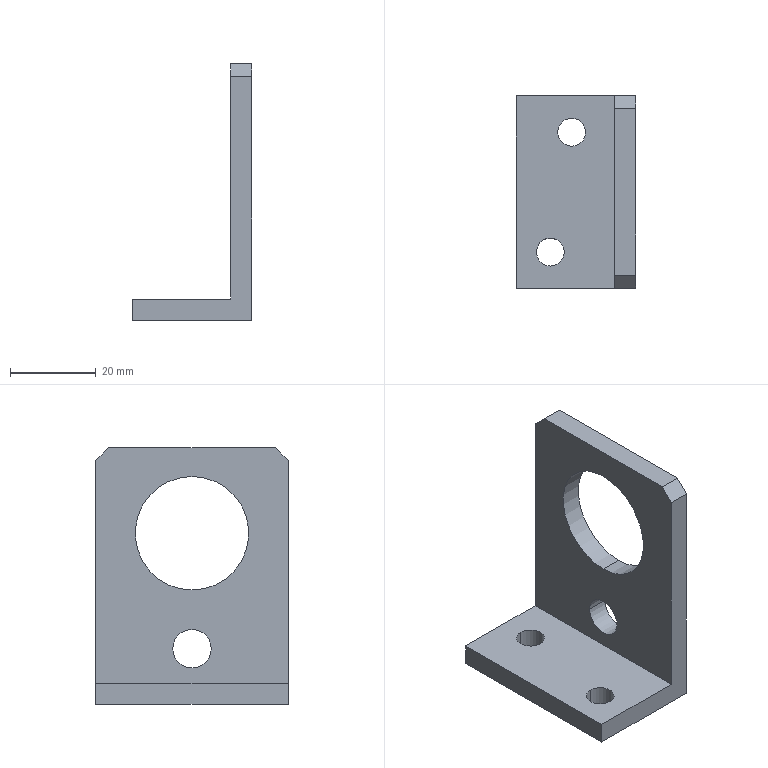Component | SolidWorks | DC-Motor-113-1 | 1 solid | 18 faces | box 28 x 45 x 60 mm | volume 15222 mm3 | plane 10 | cylinder 8 | commonest cylinder face diameters 6.5 x4 9 x2 26.5 x2
build123d program:
from build123d import *

# Parameters (mm, degrees)
BOSS_EXTRUDE1_DEPTH          = 22.5
SKETCH4_R                    = 13.25
CUT_EXTRUDE1_DEPTH           = 42
CHAMFER1_SIZE                = 3
F_6_5_6_5_DIAMETER_HOLE1_D   = 6.5
F_9_0_9_DIAMETER_HOLE1_D     = 9
F_9_0_9_DIAMETER_HOLE1_DEPTH = 12.4
F_9_0_9_DIAMETER_HOLE1_TIP   = 2.704


with BuildPart() as part:
    # Sketch1 → Boss-Extrude1 (new, symmetric)
    with BuildSketch(Plane.XY):
        Polygon((0, 60), (0, 0), (28, 0), (28, 5), (5, 5), (5, 60), align=None)
    extrude(amount=BOSS_EXTRUDE1_DEPTH, both=True)

    # Sketch4 → Cut-Extrude1 (cut)
    with BuildSketch(Plane(origin=(5, 0, 0), x_dir=(0, 0, -1), z_dir=(1, 0, 0))):
        with Locations(Location((0, 40, 0), (0, 0, 90))):
            Circle(SKETCH4_R)
    extrude(amount=-CUT_EXTRUDE1_DEPTH, mode=Mode.SUBTRACT)

    # Chamfer1
    chamfer1_edges = [part.edges().sort_by_distance(p)[0] for p in [
        (2.5, 60, 22.5),
        (2.5, 60, -22.5),
    ]]
    chamfer(chamfer1_edges, length=CHAMFER1_SIZE)

    # 6.5 _6.5_ Diameter Hole1 (through all)
    with Locations(Plane(origin=(0, 5, 0), x_dir=(1, 0, 0), z_dir=(0, 1, 0))):
        with Locations((20, 14), (15, -14)):
            Hole(F_6_5_6_5_DIAMETER_HOLE1_D / 2)

    # 9.0 _9_ Diameter Hole1
    with Locations(Plane(origin=(5, 0, 0), x_dir=(0, 0, -1), z_dir=(1, 0, 0))):
        with Locations((0, 13)):
            Hole(F_9_0_9_DIAMETER_HOLE1_D / 2, depth=F_9_0_9_DIAMETER_HOLE1_DEPTH)
            with Locations((0, 0, -(F_9_0_9_DIAMETER_HOLE1_DEPTH + F_9_0_9_DIAMETER_HOLE1_TIP / 2))):  # 118° drill point
                Cone(0, F_9_0_9_DIAMETER_HOLE1_D / 2, F_9_0_9_DIAMETER_HOLE1_TIP, mode=Mode.SUBTRACT)


solid = part.part

# Placed as in the assembly
solid = solid.moved(Location((-459.792, 14.301, -420), (-90, 0, 180)))
STEP:
#1=CARTESIAN_POINT('',(-18.102,0.7402,-16.024));
#2=VERTEX_POINT('',#1);
#3=CARTESIAN_POINT('',(-18.102,0.3859,-16.024));
#4=VERTEX_POINT('',#3);
#5=CARTESIAN_POINT('',(-18.102,0.563,-16.024));
#6=DIRECTION('',(-1.,-0.,-0.));
#7=DIRECTION('',(0.,-0.,1.));
#8=AXIS2_PLACEMENT_3D('',#5,#6,#7);
#9=CIRCLE('',#8,0.1772);
#10=EDGE_CURVE('',#2,#4,#9,.T.);
#11=ORIENTED_EDGE('',*,*,#10,.F.);
#12=CARTESIAN_POINT('',(-18.299,0.7402,-16.024));
#13=VERTEX_POINT('',#12);
#14=CARTESIAN_POINT('',(-18.299,0.7402,-16.024));
#15=DIRECTION('',(-1.,-0.,-0.));
#16=VECTOR('',#15,39.37);
#17=LINE('',#14,#16);
#18=EDGE_CURVE('',#2,#13,#17,.T.);
#19=ORIENTED_EDGE('',*,*,#18,.T.);
#20=CARTESIAN_POINT('',(-18.299,0.3859,-16.024));
#21=VERTEX_POINT('',#20);
#22=CARTESIAN_POINT('',(-18.299,0.563,-16.024));
#23=DIRECTION('',(-1.,-0.,-0.));
#24=DIRECTION('',(0.,-1.,0.));
#25=AXIS2_PLACEMENT_3D('',#22,#23,#24);
#26=CIRCLE('',#25,0.1772);
#27=EDGE_CURVE('',#13,#21,#26,.T.);
#28=ORIENTED_EDGE('',*,*,#27,.T.);
#29=CARTESIAN_POINT('',(-18.299,0.3859,-16.024));
#30=DIRECTION('',(-1.,-0.,-0.));
#31=VECTOR('',#30,39.37);
#32=LINE('',#29,#31);
#33=EDGE_CURVE('',#4,#21,#32,.T.);
#34=ORIENTED_EDGE('',*,*,#33,.F.);
#35=EDGE_LOOP('',(#11,#19,#28,#34));
#36=FACE_OUTER_BOUND('',#35,.T.);
#37=CARTESIAN_POINT('',(-18.299,0.563,-16.024));
#38=DIRECTION('',(-1.,-0.,-0.));
#39=DIRECTION('',(0.,-1.,0.));
#40=AXIS2_PLACEMENT_3D('',#37,#38,#39);
#41=CYLINDRICAL_SURFACE('',#40,0.1772);
#42=ADVANCED_FACE('',(#36),#41,.F.);
#43=CARTESIAN_POINT('',(-18.889,-0.1161,-16.535));
#44=VERTEX_POINT('',#43);
#45=CARTESIAN_POINT('',(-18.889,0.1398,-16.535));
#46=VERTEX_POINT('',#45);
#47=CARTESIAN_POINT('',(-18.889,0.01186,-16.535));
#48=DIRECTION('',(-0.,-0.,1.));
#49=DIRECTION('',(0.,1.,0.));
#50=AXIS2_PLACEMENT_3D('',#47,#48,#49);
#51=CIRCLE('',#50,0.128);
#52=EDGE_CURVE('',#44,#46,#51,.T.);
#53=ORIENTED_EDGE('',*,*,#52,.F.);
#54=CARTESIAN_POINT('',(-18.889,-0.1161,-16.339));
#55=VERTEX_POINT('',#54);
#56=CARTESIAN_POINT('',(-18.889,-0.1161,-16.339));
#57=DIRECTION('',(-0.,-0.,1.));
#58=VECTOR('',#57,39.37);
#59=LINE('',#56,#58);
#60=EDGE_CURVE('',#44,#55,#59,.T.);
#61=ORIENTED_EDGE('',*,*,#60,.T.);
#62=CARTESIAN_POINT('',(-18.889,0.1398,-16.339));
#63=VERTEX_POINT('',#62);
#64=CARTESIAN_POINT('',(-18.889,0.01186,-16.339));
#65=DIRECTION('',(-0.,-0.,1.));
#66=DIRECTION('',(0.,1.,0.));
#67=AXIS2_PLACEMENT_3D('',#64,#65,#66);
#68=CIRCLE('',#67,0.128);
#69=EDGE_CURVE('',#55,#63,#68,.T.);
#70=ORIENTED_EDGE('',*,*,#69,.T.);
#71=CARTESIAN_POINT('',(-18.889,0.1398,-16.339));
#72=DIRECTION('',(-0.,-0.,1.));
#73=VECTOR('',#72,39.37);
#74=LINE('',#71,#73);
#75=EDGE_CURVE('',#46,#63,#74,.T.);
#76=ORIENTED_EDGE('',*,*,#75,.F.);
#77=EDGE_LOOP('',(#53,#61,#70,#76));
#78=FACE_OUTER_BOUND('',#77,.T.);
#79=CARTESIAN_POINT('',(-18.889,0.01186,-16.339));
#80=DIRECTION('',(-0.,-0.,1.));
#81=DIRECTION('',(0.,1.,0.));
#82=AXIS2_PLACEMENT_3D('',#79,#80,#81);
#83=CYLINDRICAL_SURFACE('',#82,0.128);
#84=ADVANCED_FACE('',(#78),#83,.F.);
#85=CARTESIAN_POINT('',(-18.693,0.9863,-16.535));
#86=VERTEX_POINT('',#85);
#87=CARTESIAN_POINT('',(-18.693,1.242,-16.535));
#88=VERTEX_POINT('',#87);
#89=CARTESIAN_POINT('',(-18.693,1.114,-16.535));
#90=DIRECTION('',(-0.,-0.,1.));
#91=DIRECTION('',(0.,1.,0.));
#92=AXIS2_PLACEMENT_3D('',#89,#90,#91);
#93=CIRCLE('',#92,0.128);
#94=EDGE_CURVE('',#86,#88,#93,.T.);
#95=ORIENTED_EDGE('',*,*,#94,.F.);
#96=CARTESIAN_POINT('',(-18.693,0.9863,-16.339));
#97=VERTEX_POINT('',#96);
#98=CARTESIAN_POINT('',(-18.693,0.9863,-16.339));
#99=DIRECTION('',(-0.,-0.,1.));
#100=VECTOR('',#99,39.37);
#101=LINE('',#98,#100);
#102=EDGE_CURVE('',#86,#97,#101,.T.);
#103=ORIENTED_EDGE('',*,*,#102,.T.);
#104=CARTESIAN_POINT('',(-18.693,1.242,-16.339));
#105=VERTEX_POINT('',#104);
#106=CARTESIAN_POINT('',(-18.693,1.114,-16.339));
#107=DIRECTION('',(-0.,-0.,1.));
#108=DIRECTION('',(0.,1.,0.));
#109=AXIS2_PLACEMENT_3D('',#106,#107,#108);
#110=CIRCLE('',#109,0.128);
#111=EDGE_CURVE('',#97,#105,#110,.T.);
#112=ORIENTED_EDGE('',*,*,#111,.T.);
#113=CARTESIAN_POINT('',(-18.693,1.242,-16.339));
#114=DIRECTION('',(-0.,-0.,1.));
#115=VECTOR('',#114,39.37);
#116=LINE('',#113,#115);
#117=EDGE_CURVE('',#88,#105,#116,.T.);
#118=ORIENTED_EDGE('',*,*,#117,.F.);
#119=EDGE_LOOP('',(#95,#103,#112,#118));
#120=FACE_OUTER_BOUND('',#119,.T.);
#121=CARTESIAN_POINT('',(-18.693,1.114,-16.339));
#122=DIRECTION('',(-0.,-0.,1.));
#123=DIRECTION('',(0.,1.,0.));
#124=AXIS2_PLACEMENT_3D('',#121,#122,#123);
#125=CYLINDRICAL_SURFACE('',#124,0.128);
#126=ADVANCED_FACE('',(#120),#125,.F.);
#127=CARTESIAN_POINT('',(-18.102,0.563,-15.482));
#128=VERTEX_POINT('',#127);
#129=CARTESIAN_POINT('',(-18.102,0.563,-14.439));
#130=VERTEX_POINT('',#129);
#131=CARTESIAN_POINT('',(-18.102,0.563,-14.961));
#132=DIRECTION('',(-1.,-0.,-0.));
#133=DIRECTION('',(0.,-0.,1.));
#134=AXIS2_PLACEMENT_3D('',#131,#132,#133);
#135=CIRCLE('',#134,0.5217);
#136=EDGE_CURVE('',#128,#130,#135,.T.);
#137=ORIENTED_EDGE('',*,*,#136,.F.);
#138=CARTESIAN_POINT('',(-18.299,0.563,-15.482));
#139=VERTEX_POINT('',#138);
#140=CARTESIAN_POINT('',(-16.645,0.563,-15.482));
#141=DIRECTION('',(-1.,-0.,-0.));
#142=VECTOR('',#141,39.37);
#143=LINE('',#140,#142);
#144=EDGE_CURVE('',#128,#139,#143,.T.);
#145=ORIENTED_EDGE('',*,*,#144,.T.);
#146=CARTESIAN_POINT('',(-18.299,0.563,-14.439));
#147=VERTEX_POINT('',#146);
#148=CARTESIAN_POINT('',(-18.299,0.563,-14.961));
#149=DIRECTION('',(-1.,-0.,-0.));
#150=DIRECTION('',(0.,-0.,1.));
#151=AXIS2_PLACEMENT_3D('',#148,#149,#150);
#152=CIRCLE('',#151,0.5217);
#153=EDGE_CURVE('',#139,#147,#152,.T.);
#154=ORIENTED_EDGE('',*,*,#153,.T.);
#155=CARTESIAN_POINT('',(-16.645,0.563,-14.439));
#156=DIRECTION('',(-1.,-0.,-0.));
#157=VECTOR('',#156,39.37);
#158=LINE('',#155,#157);
#159=EDGE_CURVE('',#130,#147,#158,.T.);
#160=ORIENTED_EDGE('',*,*,#159,.F.);
#161=EDGE_LOOP('',(#137,#145,#154,#160));
#162=FACE_OUTER_BOUND('',#161,.T.);
#163=CARTESIAN_POINT('',(-16.645,0.563,-14.961));
#164=DIRECTION('',(-1.,-0.,-0.));
#165=DIRECTION('',(0.,-0.,1.));
#166=AXIS2_PLACEMENT_3D('',#163,#164,#165);
#167=CYLINDRICAL_SURFACE('',#166,0.5217);
#168=ADVANCED_FACE('',(#162),#167,.F.);
#169=CARTESIAN_POINT('',(-18.299,1.331,-14.173));
#170=VERTEX_POINT('',#169);
#171=CARTESIAN_POINT('',(-18.299,-0.2047,-14.173));
#172=VERTEX_POINT('',#171);
#173=CARTESIAN_POINT('',(-18.299,1.449,-14.173));
#174=DIRECTION('',(0.,-1.,-0.));
#175=VECTOR('',#174,39.37);
#176=LINE('',#173,#175);
#177=EDGE_CURVE('',#170,#172,#176,.T.);
#178=ORIENTED_EDGE('',*,*,#177,.T.);
#179=CARTESIAN_POINT('',(-18.102,-0.2047,-14.173));
#180=VERTEX_POINT('',#179);
#181=CARTESIAN_POINT('',(-18.102,-0.2047,-14.173));
#182=DIRECTION('',(1.,0.,0.));
#183=VECTOR('',#182,39.37);
#184=LINE('',#181,#183);
#185=EDGE_CURVE('',#172,#180,#184,.T.);
#186=ORIENTED_EDGE('',*,*,#185,.T.);
#187=CARTESIAN_POINT('',(-18.102,1.331,-14.173));
#188=VERTEX_POINT('',#187);
#189=CARTESIAN_POINT('',(-18.102,1.449,-14.173));
#190=DIRECTION('',(0.,-1.,-0.));
#191=VECTOR('',#190,39.37);
#192=LINE('',#189,#191);
#193=EDGE_CURVE('',#188,#180,#192,.T.);
#194=ORIENTED_EDGE('',*,*,#193,.F.);
#195=CARTESIAN_POINT('',(-18.102,1.331,-14.173));
#196=DIRECTION('',(-1.,-0.,-0.));
#197=VECTOR('',#196,39.37);
#198=LINE('',#195,#197);
#199=EDGE_CURVE('',#188,#170,#198,.T.);
#200=ORIENTED_EDGE('',*,*,#199,.T.);
#201=EDGE_LOOP('',(#178,#186,#194,#200));
#202=FACE_OUTER_BOUND('',#201,.T.);
#203=CARTESIAN_POINT('',(-18.102,1.449,-14.173));
#204=DIRECTION('',(0.,0.,-1.));
#205=DIRECTION('',(0.,-1.,-0.));
#206=AXIS2_PLACEMENT_3D('',#203,#204,#205);
#207=PLANE('',#206);
#208=ADVANCED_FACE('',(#202),#207,.F.);
#209=CARTESIAN_POINT('',(-18.102,0.563,-16.024));
#210=DIRECTION('',(-1.,-0.,-0.));
#211=DIRECTION('',(0.,-0.,1.));
#212=AXIS2_PLACEMENT_3D('',#209,#210,#211);
#213=CIRCLE('',#212,0.1772);
#214=EDGE_CURVE('',#4,#2,#213,.T.);
#215=ORIENTED_EDGE('',*,*,#214,.T.);
#216=ORIENTED_EDGE('',*,*,#10,.T.);
#217=EDGE_LOOP('',(#215,#216));
#218=FACE_BOUND('',#217,.T.);
#219=CARTESIAN_POINT('',(-18.102,0.563,-14.961));
#220=DIRECTION('',(-1.,-0.,-0.));
#221=DIRECTION('',(0.,-0.,1.));
#222=AXIS2_PLACEMENT_3D('',#219,#220,#221);
#223=CIRCLE('',#222,0.5217);
#224=EDGE_CURVE('',#130,#128,#223,.T.);
#225=ORIENTED_EDGE('',*,*,#224,.T.);
#226=ORIENTED_EDGE('',*,*,#136,.T.);
#227=EDGE_LOOP('',(#225,#226));
#228=FACE_BOUND('',#227,.T.);
#229=ORIENTED_EDGE('',*,*,#193,.T.);
#230=CARTESIAN_POINT('',(-18.102,-0.3228,-14.291));
#231=VERTEX_POINT('',#230);
#232=CARTESIAN_POINT('',(-18.102,-0.2047,-14.173));
#233=DIRECTION('',(0.,-0.7071,-0.7071));
#234=VECTOR('',#233,39.37);
#235=LINE('',#232,#234);
#236=EDGE_CURVE('',#180,#231,#235,.T.);
#237=ORIENTED_EDGE('',*,*,#236,.T.);
#238=CARTESIAN_POINT('',(-18.102,-0.3228,-16.535));
#239=VERTEX_POINT('',#238);
#240=CARTESIAN_POINT('',(-18.102,-0.3228,-14.173));
#241=DIRECTION('',(0.,0.,-1.));
#242=VECTOR('',#241,39.37);
#243=LINE('',#240,#242);
#244=EDGE_CURVE('',#231,#239,#243,.T.);
#245=ORIENTED_EDGE('',*,*,#244,.T.);
#246=CARTESIAN_POINT('',(-18.102,1.449,-16.535));
#247=VERTEX_POINT('',#246);
#248=CARTESIAN_POINT('',(-18.102,1.449,-16.535));
#249=DIRECTION('',(0.,-1.,-0.));
#250=VECTOR('',#249,39.37);
#251=LINE('',#248,#250);
#252=EDGE_CURVE('',#247,#239,#251,.T.);
#253=ORIENTED_EDGE('',*,*,#252,.F.);
#254=CARTESIAN_POINT('',(-18.102,1.449,-14.291));
#255=VERTEX_POINT('',#254);
#256=CARTESIAN_POINT('',(-18.102,1.449,-14.173));
#257=DIRECTION('',(0.,0.,-1.));
#258=VECTOR('',#257,39.37);
#259=LINE('',#256,#258);
#260=EDGE_CURVE('',#255,#247,#259,.T.);
#261=ORIENTED_EDGE('',*,*,#260,.F.);
#262=CARTESIAN_POINT('',(-18.102,1.449,-14.291));
#263=DIRECTION('',(-0.,-0.7071,0.7071));
#264=VECTOR('',#263,39.37);
#265=LINE('',#262,#264);
#266=EDGE_CURVE('',#255,#188,#265,.T.);
#267=ORIENTED_EDGE('',*,*,#266,.T.);
#268=EDGE_LOOP('',(#229,#237,#245,#253,#261,#267));
#269=FACE_OUTER_BOUND('',#268,.T.);
#270=CARTESIAN_POINT('',(-18.102,1.449,-14.173));
#271=DIRECTION('',(-1.,-0.,-0.));
#272=DIRECTION('',(-0.,-0.,1.));
#273=AXIS2_PLACEMENT_3D('',#270,#271,#272);
#274=PLANE('',#273);
#275=ADVANCED_FACE('',(#218,#228,#269),#274,.F.);
#276=CARTESIAN_POINT('',(-18.889,0.01186,-16.535));
#277=DIRECTION('',(-0.,-0.,1.));
#278=DIRECTION('',(0.,1.,0.));
#279=AXIS2_PLACEMENT_3D('',#276,#277,#278);
#280=CIRCLE('',#279,0.128);
#281=EDGE_CURVE('',#46,#44,#280,.T.);
#282=ORIENTED_EDGE('',*,*,#281,.T.);
#283=ORIENTED_EDGE('',*,*,#52,.T.);
#284=EDGE_LOOP('',(#282,#283));
#285=FACE_BOUND('',#284,.T.);
#286=CARTESIAN_POINT('',(-18.693,1.114,-16.535));
#287=DIRECTION('',(-0.,-0.,1.));
#288=DIRECTION('',(0.,1.,0.));
#289=AXIS2_PLACEMENT_3D('',#286,#287,#288);
#290=CIRCLE('',#289,0.128);
#291=EDGE_CURVE('',#88,#86,#290,.T.);
#292=ORIENTED_EDGE('',*,*,#291,.T.);
#293=ORIENTED_EDGE('',*,*,#94,.T.);
#294=EDGE_LOOP('',(#292,#293));
#295=FACE_BOUND('',#294,.T.);
#296=CARTESIAN_POINT('',(-19.204,-0.3228,-16.535));
#297=VERTEX_POINT('',#296);
#298=CARTESIAN_POINT('',(-18.102,-0.3228,-16.535));
#299=DIRECTION('',(-1.,-0.,-0.));
#300=VECTOR('',#299,39.37);
#301=LINE('',#298,#300);
#302=EDGE_CURVE('',#239,#297,#301,.T.);
#303=ORIENTED_EDGE('',*,*,#302,.T.);
#304=CARTESIAN_POINT('',(-19.204,1.449,-16.535));
#305=VERTEX_POINT('',#304);
#306=CARTESIAN_POINT('',(-19.204,1.449,-16.535));
#307=DIRECTION('',(0.,-1.,-0.));
#308=VECTOR('',#307,39.37);
#309=LINE('',#306,#308);
#310=EDGE_CURVE('',#305,#297,#309,.T.);
#311=ORIENTED_EDGE('',*,*,#310,.F.);
#312=CARTESIAN_POINT('',(-18.102,1.449,-16.535));
#313=DIRECTION('',(-1.,-0.,-0.));
#314=VECTOR('',#313,39.37);
#315=LINE('',#312,#314);
#316=EDGE_CURVE('',#247,#305,#315,.T.);
#317=ORIENTED_EDGE('',*,*,#316,.F.);
#318=ORIENTED_EDGE('',*,*,#252,.T.);
#319=EDGE_LOOP('',(#303,#311,#317,#318));
#320=FACE_OUTER_BOUND('',#319,.T.);
#321=CARTESIAN_POINT('',(-18.102,1.449,-16.535));
#322=DIRECTION('',(-0.,-0.,1.));
#323=DIRECTION('',(-0.,1.,0.));
#324=AXIS2_PLACEMENT_3D('',#321,#322,#323);
#325=PLANE('',#324);
#326=ADVANCED_FACE('',(#285,#295,#320),#325,.F.);
#327=CARTESIAN_POINT('',(-19.204,-0.3228,-16.339));
#328=VERTEX_POINT('',#327);
#329=CARTESIAN_POINT('',(-19.204,-0.3228,-16.339));
#330=DIRECTION('',(-0.,-0.,1.));
#331=VECTOR('',#330,39.37);
#332=LINE('',#329,#331);
#333=EDGE_CURVE('',#297,#328,#332,.T.);
#334=ORIENTED_EDGE('',*,*,#333,.T.);
#335=CARTESIAN_POINT('',(-19.204,1.449,-16.339));
#336=VERTEX_POINT('',#335);
#337=CARTESIAN_POINT('',(-19.204,1.449,-16.339));
#338=DIRECTION('',(0.,-1.,-0.));
#339=VECTOR('',#338,39.37);
#340=LINE('',#337,#339);
#341=EDGE_CURVE('',#336,#328,#340,.T.);
#342=ORIENTED_EDGE('',*,*,#341,.F.);
#343=CARTESIAN_POINT('',(-19.204,1.449,-16.339));
#344=DIRECTION('',(-0.,-0.,1.));
#345=VECTOR('',#344,39.37);
#346=LINE('',#343,#345);
#347=EDGE_CURVE('',#305,#336,#346,.T.);
#348=ORIENTED_EDGE('',*,*,#347,.F.);
#349=ORIENTED_EDGE('',*,*,#310,.T.);
#350=EDGE_LOOP('',(#334,#342,#348,#349));
#351=FACE_OUTER_BOUND('',#350,.T.);
#352=CARTESIAN_POINT('',(-19.204,1.449,-16.339));
#353=DIRECTION('',(1.,0.,0.));
#354=DIRECTION('',(-0.,1.,0.));
#355=AXIS2_PLACEMENT_3D('',#352,#353,#354);
#356=PLANE('',#355);
#357=ADVANCED_FACE('',(#351),#356,.F.);
#358=CARTESIAN_POINT('',(-18.889,0.01186,-16.339));
#359=DIRECTION('',(-0.,-0.,1.));
#360=DIRECTION('',(0.,1.,0.));
#361=AXIS2_PLACEMENT_3D('',#358,#359,#360);
#362=CIRCLE('',#361,0.128);
#363=EDGE_CURVE('',#63,#55,#362,.T.);
#364=ORIENTED_EDGE('',*,*,#363,.F.);
#365=ORIENTED_EDGE('',*,*,#69,.F.);
#366=EDGE_LOOP('',(#364,#365));
#367=FACE_BOUND('',#366,.T.);
#368=CARTESIAN_POINT('',(-18.693,1.114,-16.339));
#369=DIRECTION('',(-0.,-0.,1.));
#370=DIRECTION('',(0.,1.,0.));
#371=AXIS2_PLACEMENT_3D('',#368,#369,#370);
#372=CIRCLE('',#371,0.128);
#373=EDGE_CURVE('',#105,#97,#372,.T.);
#374=ORIENTED_EDGE('',*,*,#373,.F.);
#375=ORIENTED_EDGE('',*,*,#111,.F.);
#376=EDGE_LOOP('',(#374,#375));
#377=FACE_BOUND('',#376,.T.);
#378=CARTESIAN_POINT('',(-18.299,-0.3228,-16.339));
#379=VERTEX_POINT('',#378);
#380=CARTESIAN_POINT('',(-18.299,-0.3228,-16.339));
#381=DIRECTION('',(1.,0.,0.));
#382=VECTOR('',#381,39.37);
#383=LINE('',#380,#382);
#384=EDGE_CURVE('',#328,#379,#383,.T.);
#385=ORIENTED_EDGE('',*,*,#384,.T.);
#386=CARTESIAN_POINT('',(-18.299,1.449,-16.339));
#387=VERTEX_POINT('',#386);
#388=CARTESIAN_POINT('',(-18.299,1.449,-16.339));
#389=DIRECTION('',(0.,-1.,-0.));
#390=VECTOR('',#389,39.37);
#391=LINE('',#388,#390);
#392=EDGE_CURVE('',#387,#379,#391,.T.);
#393=ORIENTED_EDGE('',*,*,#392,.F.);
#394=CARTESIAN_POINT('',(-18.299,1.449,-16.339));
#395=DIRECTION('',(1.,0.,0.));
#396=VECTOR('',#395,39.37);
#397=LINE('',#394,#396);
#398=EDGE_CURVE('',#336,#387,#397,.T.);
#399=ORIENTED_EDGE('',*,*,#398,.F.);
#400=ORIENTED_EDGE('',*,*,#341,.T.);
#401=EDGE_LOOP('',(#385,#393,#399,#400));
#402=FACE_OUTER_BOUND('',#401,.T.);
#403=CARTESIAN_POINT('',(-18.299,1.449,-16.339));
#404=DIRECTION('',(0.,0.,-1.));
#405=DIRECTION('',(0.,-1.,-0.));
#406=AXIS2_PLACEMENT_3D('',#403,#404,#405);
#407=PLANE('',#406);
#408=ADVANCED_FACE('',(#367,#377,#402),#407,.F.);
#409=CARTESIAN_POINT('',(-18.299,0.563,-16.024));
#410=DIRECTION('',(-1.,-0.,-0.));
#411=DIRECTION('',(0.,-1.,0.));
#412=AXIS2_PLACEMENT_3D('',#409,#410,#411);
#413=CIRCLE('',#412,0.1772);
#414=EDGE_CURVE('',#21,#13,#413,.T.);
#415=ORIENTED_EDGE('',*,*,#414,.F.);
#416=ORIENTED_EDGE('',*,*,#27,.F.);
#417=EDGE_LOOP('',(#415,#416));
#418=FACE_BOUND('',#417,.T.);
#419=CARTESIAN_POINT('',(-18.299,0.563,-14.961));
#420=DIRECTION('',(-1.,-0.,-0.));
#421=DIRECTION('',(0.,-0.,1.));
#422=AXIS2_PLACEMENT_3D('',#419,#420,#421);
#423=CIRCLE('',#422,0.5217);
#424=EDGE_CURVE('',#147,#139,#423,.T.);
#425=ORIENTED_EDGE('',*,*,#424,.F.);
#426=ORIENTED_EDGE('',*,*,#153,.F.);
#427=EDGE_LOOP('',(#425,#426));
#428=FACE_BOUND('',#427,.T.);
#429=CARTESIAN_POINT('',(-18.299,-0.3228,-14.291));
#430=VERTEX_POINT('',#429);
#431=CARTESIAN_POINT('',(-18.299,-0.3228,-14.173));
#432=DIRECTION('',(-0.,-0.,1.));
#433=VECTOR('',#432,39.37);
#434=LINE('',#431,#433);
#435=EDGE_CURVE('',#379,#430,#434,.T.);
#436=ORIENTED_EDGE('',*,*,#435,.T.);
#437=CARTESIAN_POINT('',(-18.299,-0.2047,-14.173));
#438=DIRECTION('',(-0.,0.7071,0.7071));
#439=VECTOR('',#438,39.37);
#440=LINE('',#437,#439);
#441=EDGE_CURVE('',#430,#172,#440,.T.);
#442=ORIENTED_EDGE('',*,*,#441,.T.);
#443=ORIENTED_EDGE('',*,*,#177,.F.);
#444=CARTESIAN_POINT('',(-18.299,1.449,-14.291));
#445=VERTEX_POINT('',#444);
#446=CARTESIAN_POINT('',(-18.299,1.449,-14.291));
#447=DIRECTION('',(0.,0.7071,-0.7071));
#448=VECTOR('',#447,39.37);
#449=LINE('',#446,#448);
#450=EDGE_CURVE('',#170,#445,#449,.T.);
#451=ORIENTED_EDGE('',*,*,#450,.T.);
#452=CARTESIAN_POINT('',(-18.299,1.449,-14.173));
#453=DIRECTION('',(-0.,-0.,1.));
#454=VECTOR('',#453,39.37);
#455=LINE('',#452,#454);
#456=EDGE_CURVE('',#387,#445,#455,.T.);
#457=ORIENTED_EDGE('',*,*,#456,.F.);
#458=ORIENTED_EDGE('',*,*,#392,.T.);
#459=EDGE_LOOP('',(#436,#442,#443,#451,#457,#458));
#460=FACE_OUTER_BOUND('',#459,.T.);
#461=CARTESIAN_POINT('',(-18.299,1.449,-14.173));
#462=DIRECTION('',(1.,0.,0.));
#463=DIRECTION('',(0.,0.,-1.));
#464=AXIS2_PLACEMENT_3D('',#461,#462,#463);
#465=PLANE('',#464);
#466=ADVANCED_FACE('',(#418,#428,#460),#465,.F.);
#467=ORIENTED_EDGE('',*,*,#456,.T.);
#468=CARTESIAN_POINT('',(-18.102,1.449,-14.291));
#469=DIRECTION('',(1.,0.,0.));
#470=VECTOR('',#469,39.37);
#471=LINE('',#468,#470);
#472=EDGE_CURVE('',#445,#255,#471,.T.);
#473=ORIENTED_EDGE('',*,*,#472,.T.);
#474=ORIENTED_EDGE('',*,*,#260,.T.);
#475=ORIENTED_EDGE('',*,*,#316,.T.);
#476=ORIENTED_EDGE('',*,*,#347,.T.);
#477=ORIENTED_EDGE('',*,*,#398,.T.);
#478=EDGE_LOOP('',(#467,#473,#474,#475,#476,#477));
#479=FACE_OUTER_BOUND('',#478,.T.);
#480=CARTESIAN_POINT('',(-18.102,1.449,-16.535));
#481=DIRECTION('',(0.,-1.,-0.));
#482=DIRECTION('',(1.,0.,0.));
#483=AXIS2_PLACEMENT_3D('',#480,#481,#482);
#484=PLANE('',#483);
#485=ADVANCED_FACE('',(#479),#484,.F.);
#486=ORIENTED_EDGE('',*,*,#244,.F.);
#487=CARTESIAN_POINT('',(-18.299,-0.3228,-14.291));
#488=DIRECTION('',(-1.,-0.,-0.));
#489=VECTOR('',#488,39.37);
#490=LINE('',#487,#489);
#491=EDGE_CURVE('',#231,#430,#490,.T.);
#492=ORIENTED_EDGE('',*,*,#491,.T.);
#493=ORIENTED_EDGE('',*,*,#435,.F.);
#494=ORIENTED_EDGE('',*,*,#384,.F.);
#495=ORIENTED_EDGE('',*,*,#333,.F.);
#496=ORIENTED_EDGE('',*,*,#302,.F.);
#497=EDGE_LOOP('',(#486,#492,#493,#494,#495,#496));
#498=FACE_OUTER_BOUND('',#497,.T.);
#499=CARTESIAN_POINT('',(-18.102,-0.3228,-16.535));
#500=DIRECTION('',(0.,-1.,-0.));
#501=DIRECTION('',(1.,0.,0.));
#502=AXIS2_PLACEMENT_3D('',#499,#500,#501);
#503=PLANE('',#502);
#504=ADVANCED_FACE('',(#498),#503,.T.);
#505=ORIENTED_EDGE('',*,*,#144,.F.);
#506=ORIENTED_EDGE('',*,*,#224,.F.);
#507=ORIENTED_EDGE('',*,*,#159,.T.);
#508=ORIENTED_EDGE('',*,*,#424,.T.);
#509=EDGE_LOOP('',(#505,#506,#507,#508));
#510=FACE_OUTER_BOUND('',#509,.T.);
#511=CARTESIAN_POINT('',(-16.645,0.563,-14.961));
#512=DIRECTION('',(-1.,-0.,-0.));
#513=DIRECTION('',(0.,-0.,1.));
#514=AXIS2_PLACEMENT_3D('',#511,#512,#513);
#515=CYLINDRICAL_SURFACE('',#514,0.5217);
#516=ADVANCED_FACE('',(#510),#515,.F.);
#517=ORIENTED_EDGE('',*,*,#441,.F.);
#518=ORIENTED_EDGE('',*,*,#491,.F.);
#519=ORIENTED_EDGE('',*,*,#236,.F.);
#520=ORIENTED_EDGE('',*,*,#185,.F.);
#521=EDGE_LOOP('',(#517,#518,#519,#520));
#522=FACE_OUTER_BOUND('',#521,.T.);
#523=CARTESIAN_POINT('',(-18.102,-0.2047,-14.173));
#524=DIRECTION('',(-0.,-0.7071,0.7071));
#525=DIRECTION('',(-1.,-0.,-0.));
#526=AXIS2_PLACEMENT_3D('',#523,#524,#525);
#527=PLANE('',#526);
#528=ADVANCED_FACE('',(#522),#527,.T.);
#529=ORIENTED_EDGE('',*,*,#450,.F.);
#530=ORIENTED_EDGE('',*,*,#199,.F.);
#531=ORIENTED_EDGE('',*,*,#266,.F.);
#532=ORIENTED_EDGE('',*,*,#472,.F.);
#533=EDGE_LOOP('',(#529,#530,#531,#532));
#534=FACE_OUTER_BOUND('',#533,.T.);
#535=CARTESIAN_POINT('',(-18.102,1.449,-14.291));
#536=DIRECTION('',(0.,-0.7071,-0.7071));
#537=DIRECTION('',(1.,0.,0.));
#538=AXIS2_PLACEMENT_3D('',#535,#536,#537);
#539=PLANE('',#538);
#540=ADVANCED_FACE('',(#534),#539,.F.);
#541=ORIENTED_EDGE('',*,*,#102,.F.);
#542=ORIENTED_EDGE('',*,*,#291,.F.);
#543=ORIENTED_EDGE('',*,*,#117,.T.);
#544=ORIENTED_EDGE('',*,*,#373,.T.);
#545=EDGE_LOOP('',(#541,#542,#543,#544));
#546=FACE_OUTER_BOUND('',#545,.T.);
#547=CARTESIAN_POINT('',(-18.693,1.114,-16.339));
#548=DIRECTION('',(-0.,-0.,1.));
#549=DIRECTION('',(0.,1.,0.));
#550=AXIS2_PLACEMENT_3D('',#547,#548,#549);
#551=CYLINDRICAL_SURFACE('',#550,0.128);
#552=ADVANCED_FACE('',(#546),#551,.F.);
#553=ORIENTED_EDGE('',*,*,#60,.F.);
#554=ORIENTED_EDGE('',*,*,#281,.F.);
#555=ORIENTED_EDGE('',*,*,#75,.T.);
#556=ORIENTED_EDGE('',*,*,#363,.T.);
#557=EDGE_LOOP('',(#553,#554,#555,#556));
#558=FACE_OUTER_BOUND('',#557,.T.);
#559=CARTESIAN_POINT('',(-18.889,0.01186,-16.339));
#560=DIRECTION('',(-0.,-0.,1.));
#561=DIRECTION('',(0.,1.,0.));
#562=AXIS2_PLACEMENT_3D('',#559,#560,#561);
#563=CYLINDRICAL_SURFACE('',#562,0.128);
#564=ADVANCED_FACE('',(#558),#563,.F.);
#565=ORIENTED_EDGE('',*,*,#18,.F.);
#566=ORIENTED_EDGE('',*,*,#214,.F.);
#567=ORIENTED_EDGE('',*,*,#33,.T.);
#568=ORIENTED_EDGE('',*,*,#414,.T.);
#569=EDGE_LOOP('',(#565,#566,#567,#568));
#570=FACE_OUTER_BOUND('',#569,.T.);
#571=CARTESIAN_POINT('',(-18.299,0.563,-16.024));
#572=DIRECTION('',(-1.,-0.,-0.));
#573=DIRECTION('',(0.,-1.,0.));
#574=AXIS2_PLACEMENT_3D('',#571,#572,#573);
#575=CYLINDRICAL_SURFACE('',#574,0.1772);
#576=ADVANCED_FACE('',(#570),#575,.F.);
#577=CLOSED_SHELL('',(#42,#84,#126,#168,#208,#275,#326,#357,#408,#466,#485,#504,#516,#528,#540,#552,#564,#576));
#578=MANIFOLD_SOLID_BREP('',#577);
#579=CARTESIAN_POINT('',(0.,0.,0.));
#580=DIRECTION('',(0.,0.,1.));
#581=DIRECTION('',(1.,0.,0.));
#582=AXIS2_PLACEMENT_3D('',#579,#580,#581);
#583=(LENGTH_UNIT()NAMED_UNIT(*)SI_UNIT($,.METRE.));
#584=LENGTH_MEASURE_WITH_UNIT(LENGTH_MEASURE(0.0254),#583);
#585=DIMENSIONAL_EXPONENTS(1.,0.,0.,0.,0.,0.,0.);
#586=(CONVERSION_BASED_UNIT('',#584)LENGTH_UNIT()NAMED_UNIT(#585));
#587=UNCERTAINTY_MEASURE_WITH_UNIT(LENGTH_MEASURE(0.00001),#586,'','');
#588=(NAMED_UNIT(*)PLANE_ANGLE_UNIT()SI_UNIT($,.RADIAN.));
#589=(NAMED_UNIT(*)SI_UNIT($,.STERADIAN.)SOLID_ANGLE_UNIT());
#590=(GEOMETRIC_REPRESENTATION_CONTEXT(3)GLOBAL_UNCERTAINTY_ASSIGNED_CONTEXT((#587))GLOBAL_UNIT_ASSIGNED_CONTEXT((#586,#588,#589))REPRESENTATION_CONTEXT('',''));
#591=ADVANCED_BREP_SHAPE_REPRESENTATION('',(#578,#582),#590);
#592=COLOUR_RGB('',0.7922,0.8196,0.9333);
#593=FILL_AREA_STYLE_COLOUR('',#592);
#594=FILL_AREA_STYLE('',(#593));
#595=SURFACE_STYLE_FILL_AREA(#594);
#596=SURFACE_SIDE_STYLE('',(#595));
#597=SURFACE_STYLE_USAGE(.BOTH.,#596);
#598=PRESENTATION_STYLE_ASSIGNMENT((#597));
#599=STYLED_ITEM('',(#598),#578);
#600=PRESENTATION_LAYER_ASSIGNMENT('','',(#599));
#601=(LENGTH_UNIT()NAMED_UNIT(*)SI_UNIT($,.METRE.));
#602=LENGTH_MEASURE_WITH_UNIT(LENGTH_MEASURE(0.0254),#601);
#603=DIMENSIONAL_EXPONENTS(1.,0.,0.,0.,0.,0.,0.);
#604=(CONVERSION_BASED_UNIT('',#602)LENGTH_UNIT()NAMED_UNIT(#603));
#605=UNCERTAINTY_MEASURE_WITH_UNIT(LENGTH_MEASURE(0.00001),#604,'','');
#606=(NAMED_UNIT(*)PLANE_ANGLE_UNIT()SI_UNIT($,.RADIAN.));
#607=(NAMED_UNIT(*)SI_UNIT($,.STERADIAN.)SOLID_ANGLE_UNIT());
#608=(GEOMETRIC_REPRESENTATION_CONTEXT(3)GLOBAL_UNCERTAINTY_ASSIGNED_CONTEXT((#605))GLOBAL_UNIT_ASSIGNED_CONTEXT((#604,#606,#607))REPRESENTATION_CONTEXT('',''));
#609=MECHANICAL_DESIGN_GEOMETRIC_PRESENTATION_REPRESENTATION('',(#599),#608);